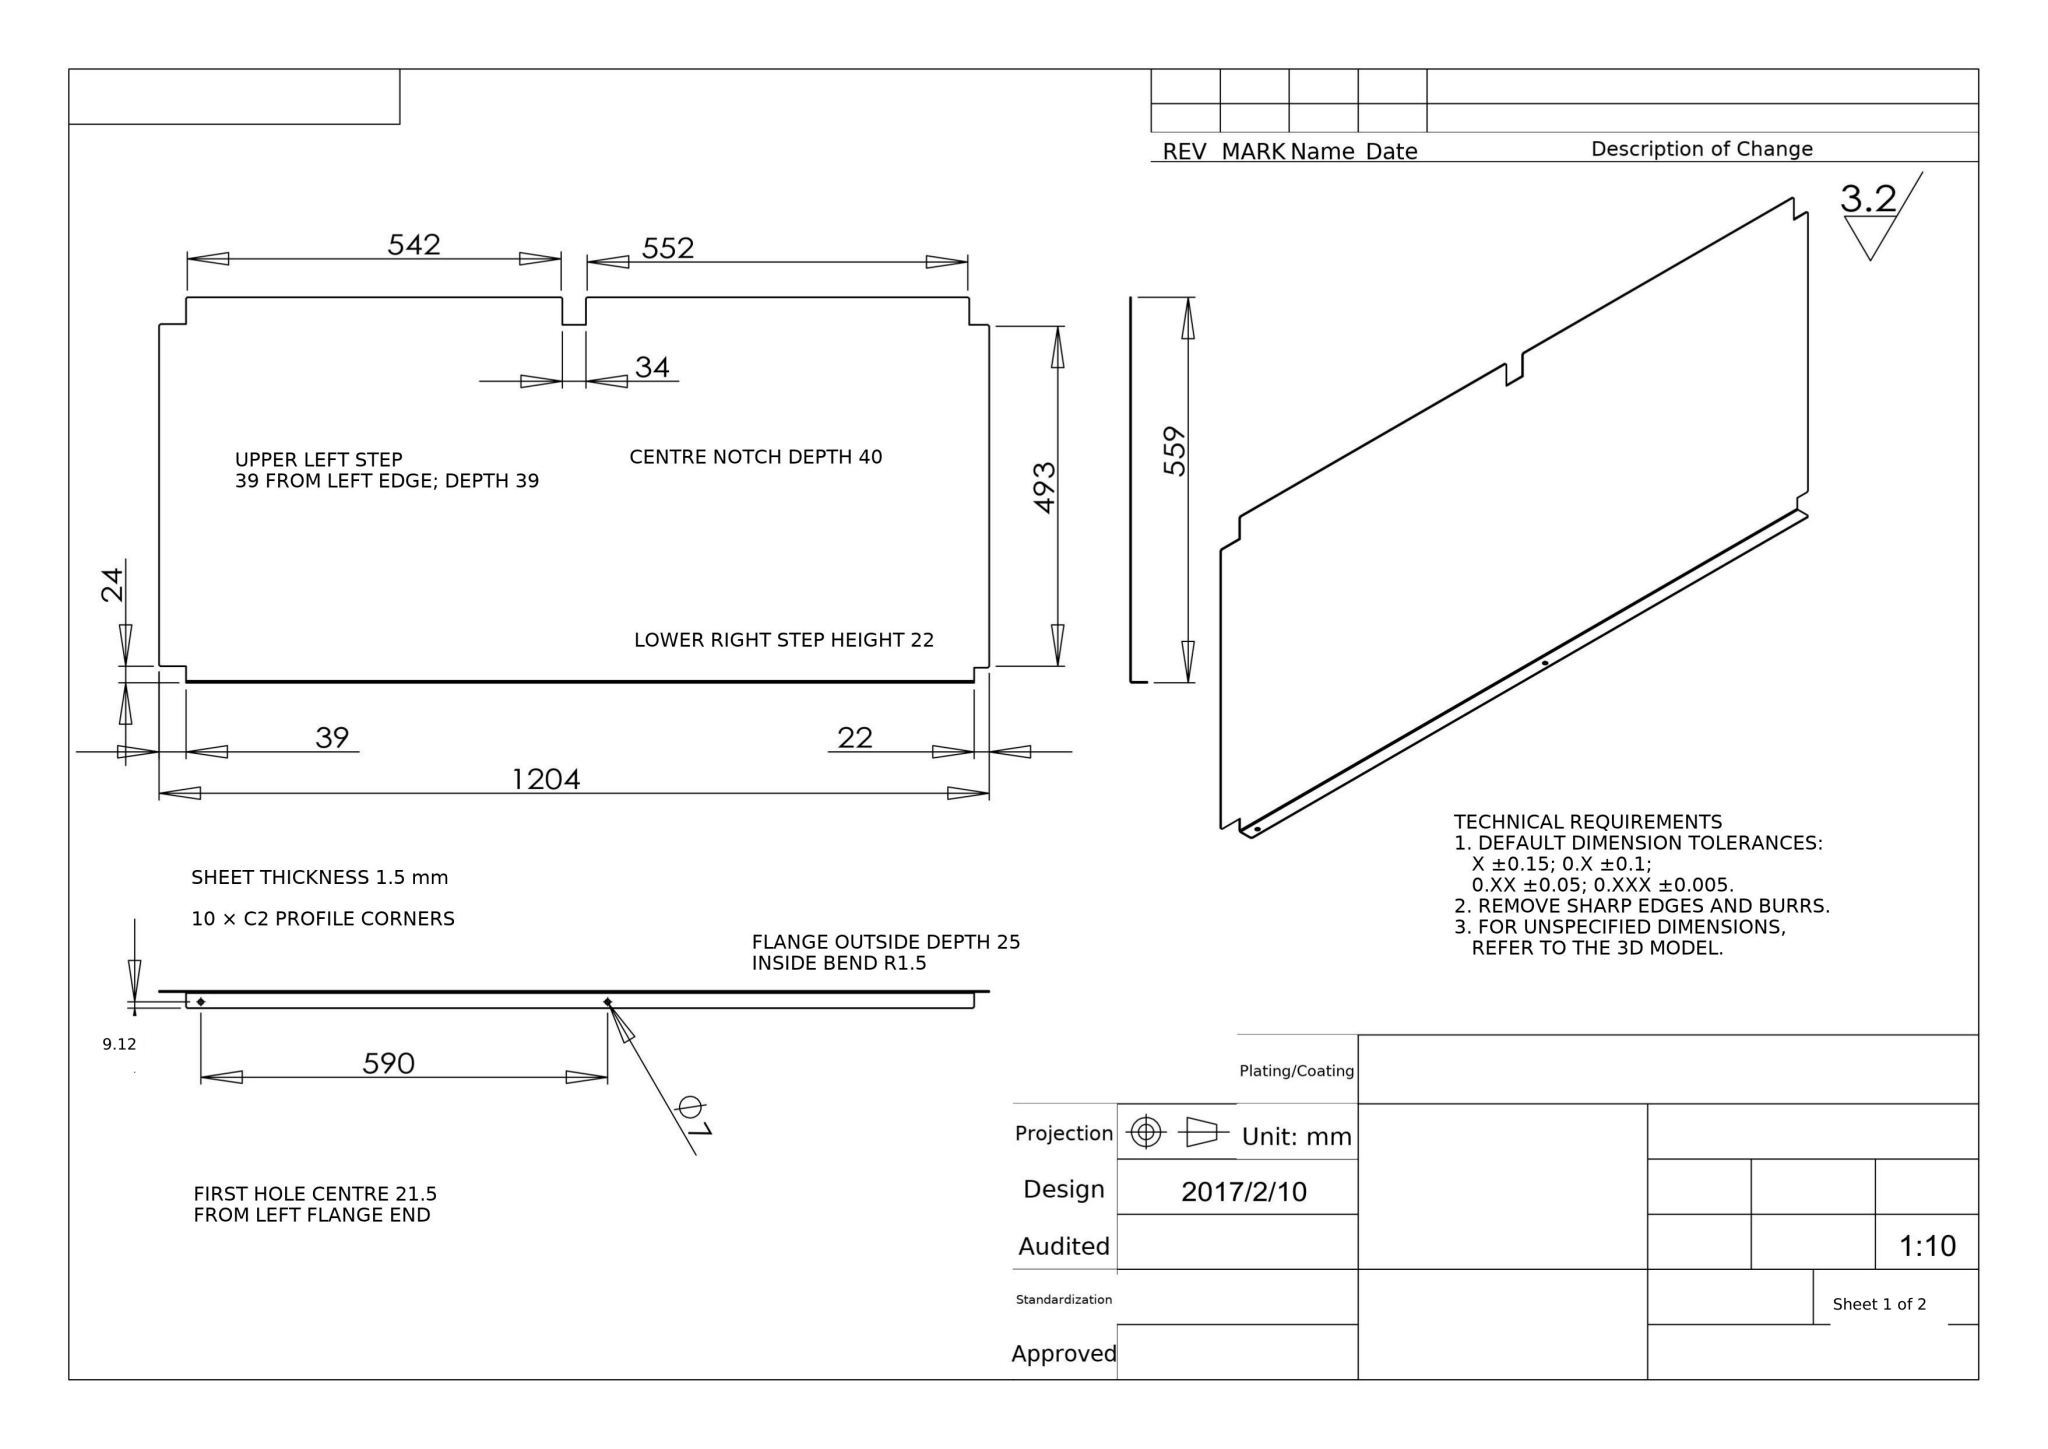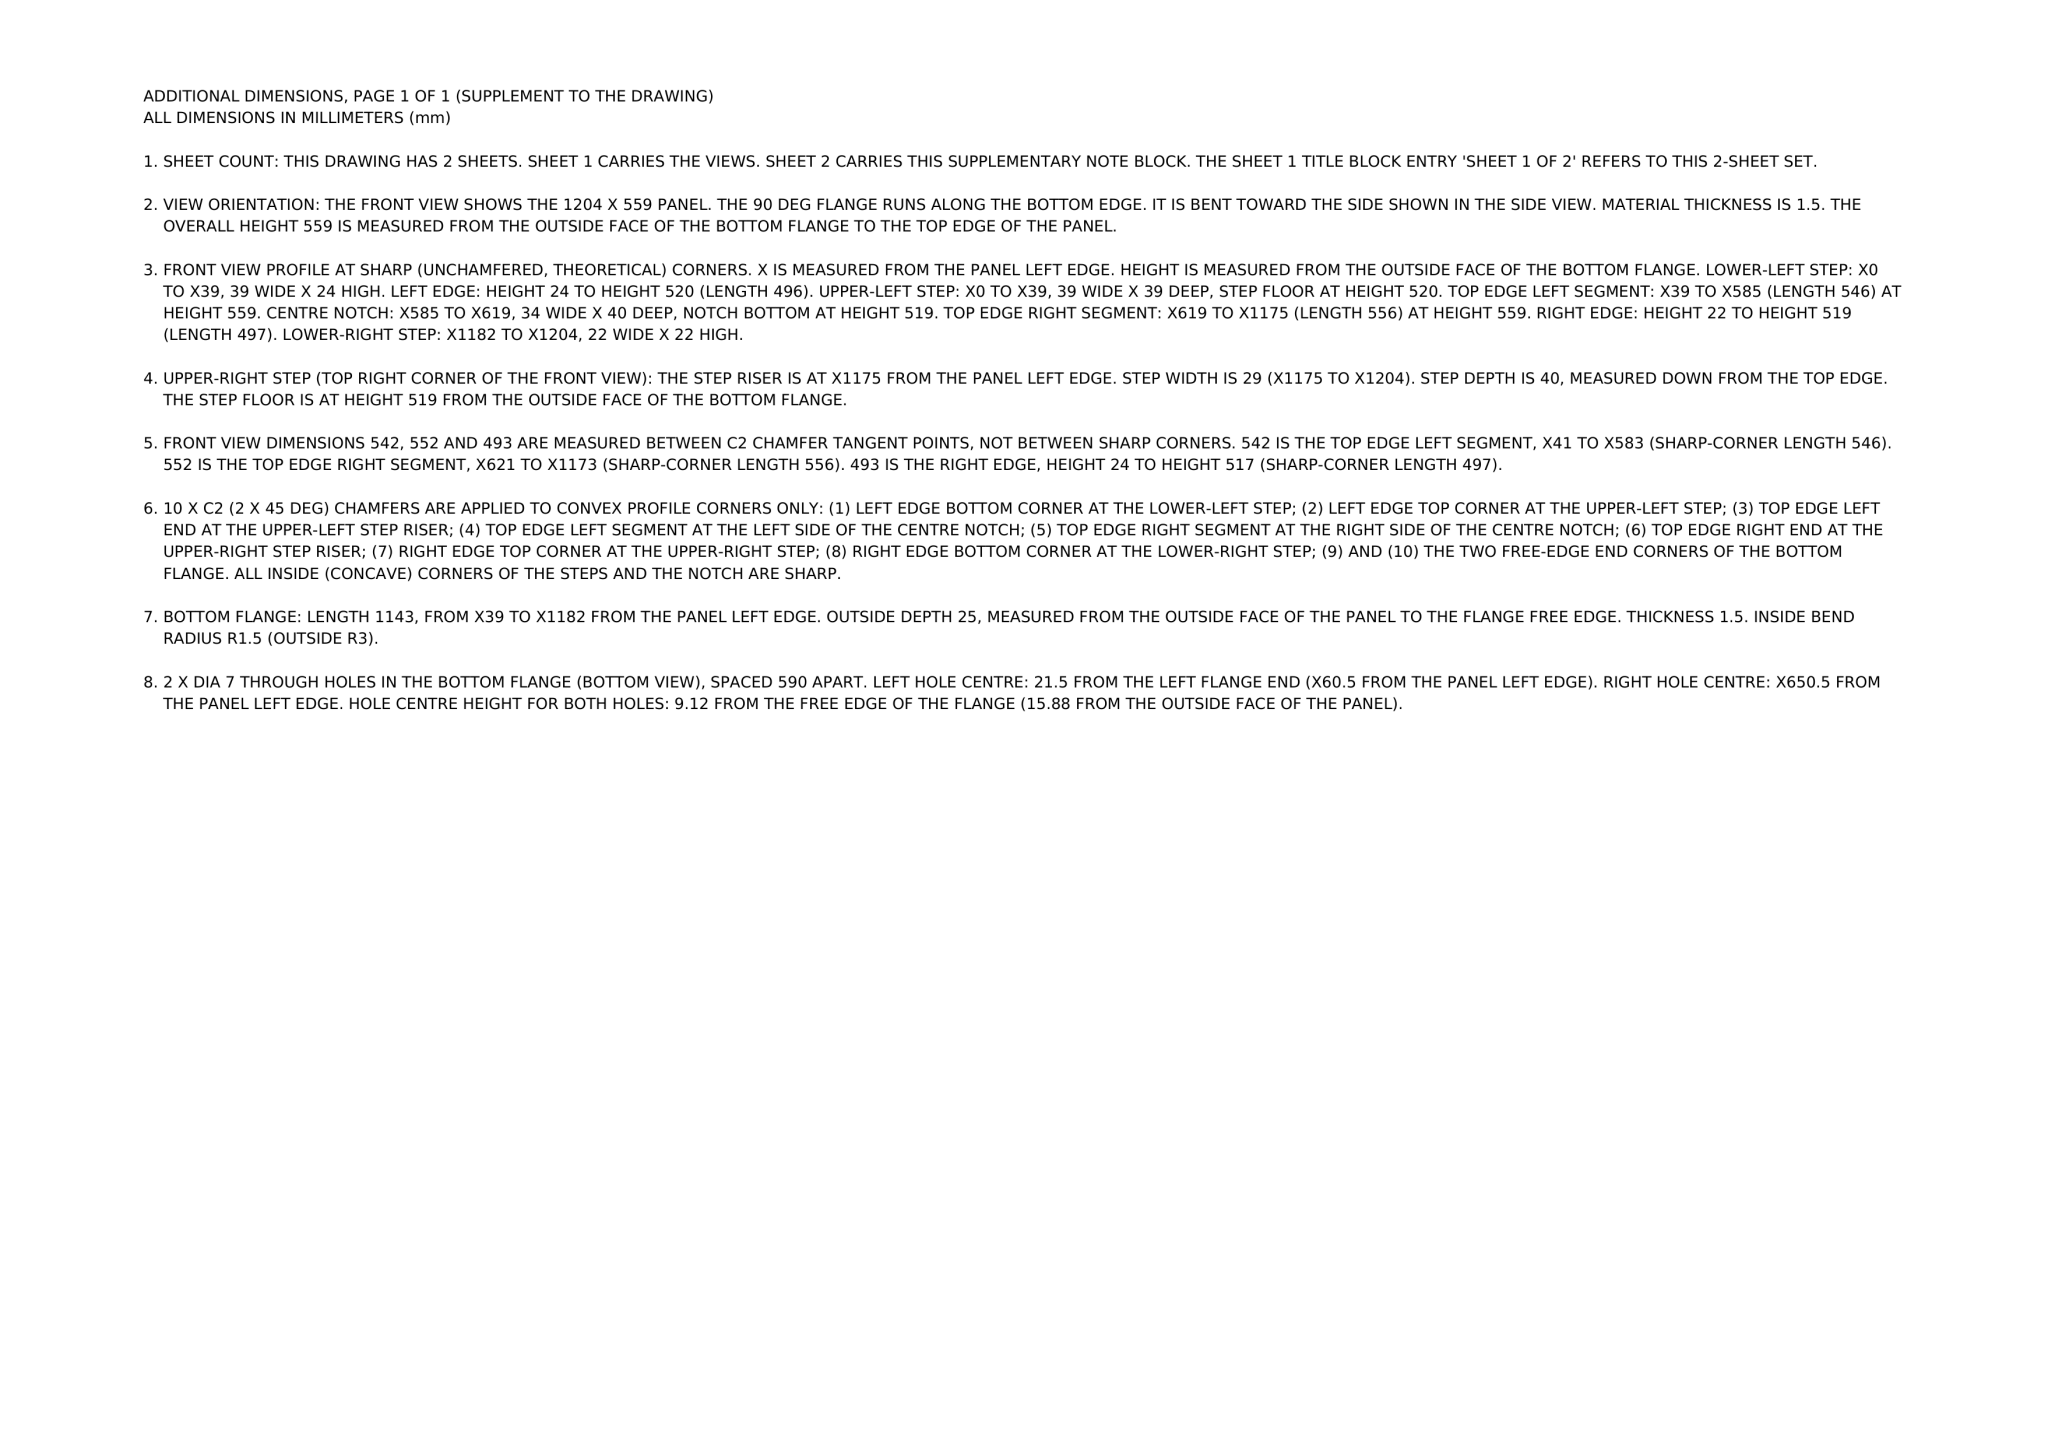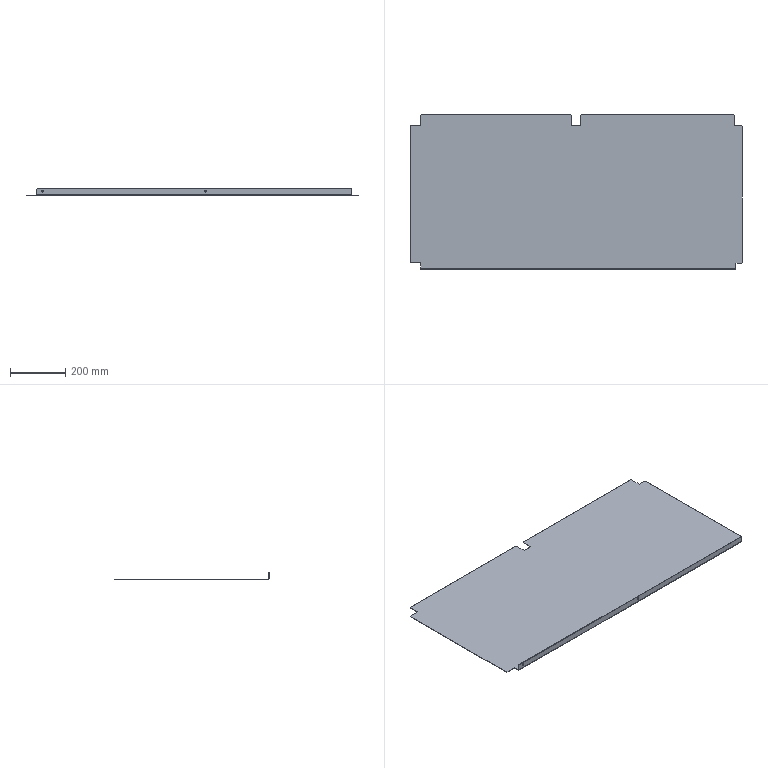Part | NX | mm | 1 solid | 40 faces | box 1204 x 559 x 25 mm | volume 1039852 mm3 | plane 34 | cylinder 6 | commonest cylinder face diameters 7 x4 6 x1 3 x1